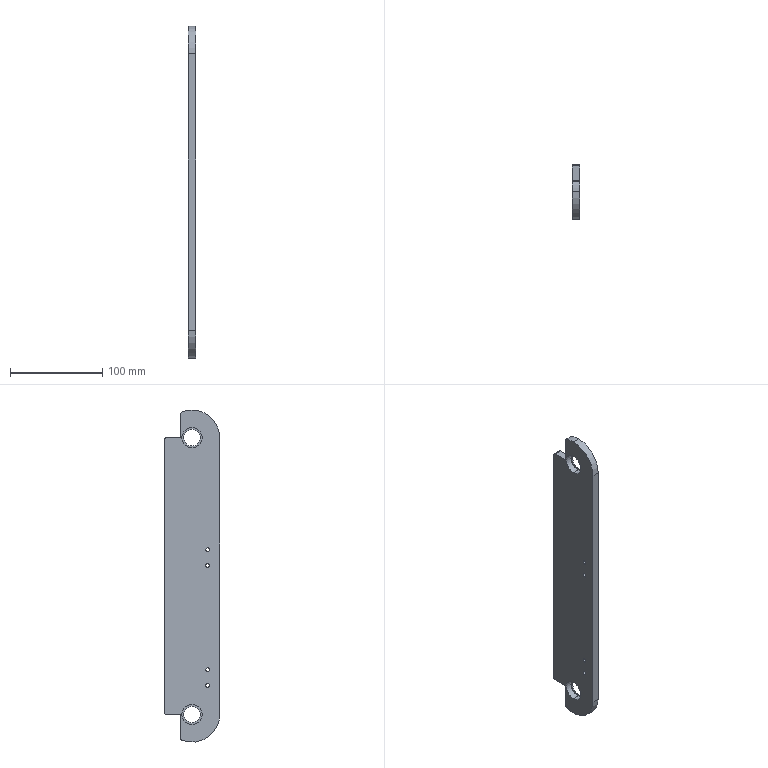Component | SolidWorks | ZHDJ-G001-2 | 1 solid | 33 faces | box 8 x 60 x 360 mm | volume 154619 mm3 | cylinder 23 | plane 10 | commonest cylinder face diameters 4.2 x8 18 x4 22 x4 4 x4 60 x3
STEP:
#1=COLOUR_RGB('',0.7922,0.8196,0.9333);
#2=FILL_AREA_STYLE_COLOUR('',#1);
#3=FILL_AREA_STYLE('',(#2));
#4=SURFACE_STYLE_FILL_AREA(#3);
#5=SURFACE_SIDE_STYLE('',(#4));
#6=SURFACE_STYLE_USAGE(.BOTH.,#5);
#7=PRESENTATION_STYLE_ASSIGNMENT((#6));
#8=CARTESIAN_POINT('',(1.772,-0.,-6.26));
#9=VERTEX_POINT('',#8);
#10=CARTESIAN_POINT('',(1.772,-0.,-5.551));
#11=VERTEX_POINT('',#10);
#12=CARTESIAN_POINT('',(1.772,-0.,-5.906));
#13=DIRECTION('',(-1.,0.,0.));
#14=DIRECTION('',(0.,0.,1.));
#15=AXIS2_PLACEMENT_3D('',#12,#13,#14);
#16=CIRCLE('',#15,0.3543);
#17=EDGE_CURVE('',#9,#11,#16,.T.);
#18=ORIENTED_EDGE('',*,*,#17,.T.);
#19=CARTESIAN_POINT('',(1.811,-0.,-5.551));
#20=VERTEX_POINT('',#19);
#21=CARTESIAN_POINT('',(1.417,-0.,-5.551));
#22=DIRECTION('',(1.,0.,0.));
#23=VECTOR('',#22,39.37);
#24=LINE('',#21,#23);
#25=EDGE_CURVE('',#11,#20,#24,.T.);
#26=ORIENTED_EDGE('',*,*,#25,.T.);
#27=CARTESIAN_POINT('',(1.811,-0.,-6.26));
#28=VERTEX_POINT('',#27);
#29=CARTESIAN_POINT('',(1.811,-0.,-5.906));
#30=DIRECTION('',(1.,0.,0.));
#31=DIRECTION('',(0.,0.,-1.));
#32=AXIS2_PLACEMENT_3D('',#29,#30,#31);
#33=CIRCLE('',#32,0.3543);
#34=EDGE_CURVE('',#20,#28,#33,.T.);
#35=ORIENTED_EDGE('',*,*,#34,.T.);
#36=CARTESIAN_POINT('',(1.417,-0.,-6.26));
#37=DIRECTION('',(1.,0.,0.));
#38=VECTOR('',#37,39.37);
#39=LINE('',#36,#38);
#40=EDGE_CURVE('',#9,#28,#39,.T.);
#41=ORIENTED_EDGE('',*,*,#40,.F.);
#42=EDGE_LOOP('',(#18,#26,#35,#41));
#43=FACE_OUTER_BOUND('',#42,.T.);
#44=CARTESIAN_POINT('',(1.417,-0.,-5.906));
#45=DIRECTION('',(1.,0.,0.));
#46=DIRECTION('',(0.,0.,-1.));
#47=AXIS2_PLACEMENT_3D('',#44,#45,#46);
#48=CYLINDRICAL_SURFACE('',#47,0.3543);
#49=ADVANCED_FACE('',(#43),#48,.F.);
#50=CARTESIAN_POINT('',(1.496,-0.6693,0.5354));
#51=VERTEX_POINT('',#50);
#52=CARTESIAN_POINT('',(1.496,-0.6693,0.3701));
#53=VERTEX_POINT('',#52);
#54=CARTESIAN_POINT('',(1.496,-0.6693,0.4528));
#55=DIRECTION('',(1.,0.,0.));
#56=DIRECTION('',(0.,0.,-1.));
#57=AXIS2_PLACEMENT_3D('',#54,#55,#56);
#58=CIRCLE('',#57,0.08268);
#59=EDGE_CURVE('',#51,#53,#58,.T.);
#60=ORIENTED_EDGE('',*,*,#59,.F.);
#61=CARTESIAN_POINT('',(1.811,-0.6693,0.5354));
#62=VERTEX_POINT('',#61);
#63=CARTESIAN_POINT('',(1.811,-0.6693,0.5354));
#64=DIRECTION('',(1.,0.,0.));
#65=VECTOR('',#64,39.37);
#66=LINE('',#63,#65);
#67=EDGE_CURVE('',#51,#62,#66,.T.);
#68=ORIENTED_EDGE('',*,*,#67,.T.);
#69=CARTESIAN_POINT('',(1.811,-0.6693,0.3701));
#70=VERTEX_POINT('',#69);
#71=CARTESIAN_POINT('',(1.811,-0.6693,0.4528));
#72=DIRECTION('',(1.,0.,0.));
#73=DIRECTION('',(0.,0.,-1.));
#74=AXIS2_PLACEMENT_3D('',#71,#72,#73);
#75=CIRCLE('',#74,0.08268);
#76=EDGE_CURVE('',#62,#70,#75,.T.);
#77=ORIENTED_EDGE('',*,*,#76,.T.);
#78=CARTESIAN_POINT('',(1.811,-0.6693,0.3701));
#79=DIRECTION('',(1.,0.,0.));
#80=VECTOR('',#79,39.37);
#81=LINE('',#78,#80);
#82=EDGE_CURVE('',#53,#70,#81,.T.);
#83=ORIENTED_EDGE('',*,*,#82,.F.);
#84=EDGE_LOOP('',(#60,#68,#77,#83));
#85=FACE_OUTER_BOUND('',#84,.T.);
#86=CARTESIAN_POINT('',(1.811,-0.6693,0.4528));
#87=DIRECTION('',(1.,0.,0.));
#88=DIRECTION('',(0.,0.,-1.));
#89=AXIS2_PLACEMENT_3D('',#86,#87,#88);
#90=CYLINDRICAL_SURFACE('',#89,0.08268);
#91=ADVANCED_FACE('',(#85),#90,.F.);
#92=CARTESIAN_POINT('',(1.496,-0.6693,1.205));
#93=VERTEX_POINT('',#92);
#94=CARTESIAN_POINT('',(1.496,-0.6693,1.039));
#95=VERTEX_POINT('',#94);
#96=CARTESIAN_POINT('',(1.496,-0.6693,1.122));
#97=DIRECTION('',(1.,0.,0.));
#98=DIRECTION('',(0.,0.,-1.));
#99=AXIS2_PLACEMENT_3D('',#96,#97,#98);
#100=CIRCLE('',#99,0.08268);
#101=EDGE_CURVE('',#93,#95,#100,.T.);
#102=ORIENTED_EDGE('',*,*,#101,.F.);
#103=CARTESIAN_POINT('',(1.811,-0.6693,1.205));
#104=VERTEX_POINT('',#103);
#105=CARTESIAN_POINT('',(1.811,-0.6693,1.205));
#106=DIRECTION('',(1.,0.,0.));
#107=VECTOR('',#106,39.37);
#108=LINE('',#105,#107);
#109=EDGE_CURVE('',#93,#104,#108,.T.);
#110=ORIENTED_EDGE('',*,*,#109,.T.);
#111=CARTESIAN_POINT('',(1.811,-0.6693,1.039));
#112=VERTEX_POINT('',#111);
#113=CARTESIAN_POINT('',(1.811,-0.6693,1.122));
#114=DIRECTION('',(1.,0.,0.));
#115=DIRECTION('',(0.,0.,-1.));
#116=AXIS2_PLACEMENT_3D('',#113,#114,#115);
#117=CIRCLE('',#116,0.08268);
#118=EDGE_CURVE('',#104,#112,#117,.T.);
#119=ORIENTED_EDGE('',*,*,#118,.T.);
#120=CARTESIAN_POINT('',(1.811,-0.6693,1.039));
#121=DIRECTION('',(1.,0.,0.));
#122=VECTOR('',#121,39.37);
#123=LINE('',#120,#122);
#124=EDGE_CURVE('',#95,#112,#123,.T.);
#125=ORIENTED_EDGE('',*,*,#124,.F.);
#126=EDGE_LOOP('',(#102,#110,#119,#125));
#127=FACE_OUTER_BOUND('',#126,.T.);
#128=CARTESIAN_POINT('',(1.811,-0.6693,1.122));
#129=DIRECTION('',(1.,0.,0.));
#130=DIRECTION('',(0.,0.,-1.));
#131=AXIS2_PLACEMENT_3D('',#128,#129,#130);
#132=CYLINDRICAL_SURFACE('',#131,0.08268);
#133=ADVANCED_FACE('',(#127),#132,.F.);
#134=CARTESIAN_POINT('',(1.496,-0.6693,-4.583));
#135=VERTEX_POINT('',#134);
#136=CARTESIAN_POINT('',(1.496,-0.6693,-4.748));
#137=VERTEX_POINT('',#136);
#138=CARTESIAN_POINT('',(1.496,-0.6693,-4.665));
#139=DIRECTION('',(1.,0.,0.));
#140=DIRECTION('',(0.,0.,-1.));
#141=AXIS2_PLACEMENT_3D('',#138,#139,#140);
#142=CIRCLE('',#141,0.08268);
#143=EDGE_CURVE('',#135,#137,#142,.T.);
#144=ORIENTED_EDGE('',*,*,#143,.F.);
#145=CARTESIAN_POINT('',(1.811,-0.6693,-4.583));
#146=VERTEX_POINT('',#145);
#147=CARTESIAN_POINT('',(1.811,-0.6693,-4.583));
#148=DIRECTION('',(1.,0.,0.));
#149=VECTOR('',#148,39.37);
#150=LINE('',#147,#149);
#151=EDGE_CURVE('',#135,#146,#150,.T.);
#152=ORIENTED_EDGE('',*,*,#151,.T.);
#153=CARTESIAN_POINT('',(1.811,-0.6693,-4.748));
#154=VERTEX_POINT('',#153);
#155=CARTESIAN_POINT('',(1.811,-0.6693,-4.665));
#156=DIRECTION('',(1.,0.,0.));
#157=DIRECTION('',(0.,0.,-1.));
#158=AXIS2_PLACEMENT_3D('',#155,#156,#157);
#159=CIRCLE('',#158,0.08268);
#160=EDGE_CURVE('',#146,#154,#159,.T.);
#161=ORIENTED_EDGE('',*,*,#160,.T.);
#162=CARTESIAN_POINT('',(1.811,-0.6693,-4.748));
#163=DIRECTION('',(1.,0.,0.));
#164=VECTOR('',#163,39.37);
#165=LINE('',#162,#164);
#166=EDGE_CURVE('',#137,#154,#165,.T.);
#167=ORIENTED_EDGE('',*,*,#166,.F.);
#168=EDGE_LOOP('',(#144,#152,#161,#167));
#169=FACE_OUTER_BOUND('',#168,.T.);
#170=CARTESIAN_POINT('',(1.811,-0.6693,-4.665));
#171=DIRECTION('',(1.,0.,0.));
#172=DIRECTION('',(0.,0.,-1.));
#173=AXIS2_PLACEMENT_3D('',#170,#171,#172);
#174=CYLINDRICAL_SURFACE('',#173,0.08268);
#175=ADVANCED_FACE('',(#169),#174,.F.);
#176=CARTESIAN_POINT('',(1.496,-0.6693,-3.913));
#177=VERTEX_POINT('',#176);
#178=CARTESIAN_POINT('',(1.496,-0.6693,-4.079));
#179=VERTEX_POINT('',#178);
#180=CARTESIAN_POINT('',(1.496,-0.6693,-3.996));
#181=DIRECTION('',(1.,0.,0.));
#182=DIRECTION('',(0.,0.,-1.));
#183=AXIS2_PLACEMENT_3D('',#180,#181,#182);
#184=CIRCLE('',#183,0.08268);
#185=EDGE_CURVE('',#177,#179,#184,.T.);
#186=ORIENTED_EDGE('',*,*,#185,.F.);
#187=CARTESIAN_POINT('',(1.811,-0.6693,-3.913));
#188=VERTEX_POINT('',#187);
#189=CARTESIAN_POINT('',(1.811,-0.6693,-3.913));
#190=DIRECTION('',(1.,0.,0.));
#191=VECTOR('',#190,39.37);
#192=LINE('',#189,#191);
#193=EDGE_CURVE('',#177,#188,#192,.T.);
#194=ORIENTED_EDGE('',*,*,#193,.T.);
#195=CARTESIAN_POINT('',(1.811,-0.6693,-4.079));
#196=VERTEX_POINT('',#195);
#197=CARTESIAN_POINT('',(1.811,-0.6693,-3.996));
#198=DIRECTION('',(1.,0.,0.));
#199=DIRECTION('',(0.,0.,-1.));
#200=AXIS2_PLACEMENT_3D('',#197,#198,#199);
#201=CIRCLE('',#200,0.08268);
#202=EDGE_CURVE('',#188,#196,#201,.T.);
#203=ORIENTED_EDGE('',*,*,#202,.T.);
#204=CARTESIAN_POINT('',(1.811,-0.6693,-4.079));
#205=DIRECTION('',(1.,0.,0.));
#206=VECTOR('',#205,39.37);
#207=LINE('',#204,#206);
#208=EDGE_CURVE('',#179,#196,#207,.T.);
#209=ORIENTED_EDGE('',*,*,#208,.F.);
#210=EDGE_LOOP('',(#186,#194,#203,#209));
#211=FACE_OUTER_BOUND('',#210,.T.);
#212=CARTESIAN_POINT('',(1.811,-0.6693,-3.996));
#213=DIRECTION('',(1.,0.,0.));
#214=DIRECTION('',(0.,0.,-1.));
#215=AXIS2_PLACEMENT_3D('',#212,#213,#214);
#216=CYLINDRICAL_SURFACE('',#215,0.08268);
#217=ADVANCED_FACE('',(#211),#216,.F.);
#218=CARTESIAN_POINT('',(1.772,0.,-5.472));
#219=VERTEX_POINT('',#218);
#220=CARTESIAN_POINT('',(1.772,0.,-6.339));
#221=VERTEX_POINT('',#220);
#222=CARTESIAN_POINT('',(1.772,0.,-5.906));
#223=DIRECTION('',(1.,0.,0.));
#224=DIRECTION('',(0.,0.,-1.));
#225=AXIS2_PLACEMENT_3D('',#222,#223,#224);
#226=CIRCLE('',#225,0.4331);
#227=EDGE_CURVE('',#219,#221,#226,.T.);
#228=ORIENTED_EDGE('',*,*,#227,.T.);
#229=CARTESIAN_POINT('',(1.496,0.,-6.339));
#230=VERTEX_POINT('',#229);
#231=CARTESIAN_POINT('',(1.772,0.,-6.339));
#232=DIRECTION('',(-1.,0.,0.));
#233=VECTOR('',#232,39.37);
#234=LINE('',#231,#233);
#235=EDGE_CURVE('',#221,#230,#234,.T.);
#236=ORIENTED_EDGE('',*,*,#235,.T.);
#237=CARTESIAN_POINT('',(1.496,0.,-5.472));
#238=VERTEX_POINT('',#237);
#239=CARTESIAN_POINT('',(1.496,0.,-5.906));
#240=DIRECTION('',(1.,0.,0.));
#241=DIRECTION('',(0.,0.,-1.));
#242=AXIS2_PLACEMENT_3D('',#239,#240,#241);
#243=CIRCLE('',#242,0.4331);
#244=EDGE_CURVE('',#238,#230,#243,.T.);
#245=ORIENTED_EDGE('',*,*,#244,.F.);
#246=CARTESIAN_POINT('',(1.772,0.,-5.472));
#247=DIRECTION('',(-1.,0.,0.));
#248=VECTOR('',#247,39.37);
#249=LINE('',#246,#248);
#250=EDGE_CURVE('',#219,#238,#249,.T.);
#251=ORIENTED_EDGE('',*,*,#250,.F.);
#252=EDGE_LOOP('',(#228,#236,#245,#251));
#253=FACE_OUTER_BOUND('',#252,.T.);
#254=CARTESIAN_POINT('',(1.772,0.,-5.906));
#255=DIRECTION('',(-1.,0.,0.));
#256=DIRECTION('',(0.,0.,1.));
#257=AXIS2_PLACEMENT_3D('',#254,#255,#256);
#258=CYLINDRICAL_SURFACE('',#257,0.4331);
#259=ADVANCED_FACE('',(#253),#258,.F.);
#260=CARTESIAN_POINT('',(1.772,0.,5.472));
#261=VERTEX_POINT('',#260);
#262=CARTESIAN_POINT('',(1.772,0.,6.339));
#263=VERTEX_POINT('',#262);
#264=CARTESIAN_POINT('',(1.772,0.,5.906));
#265=DIRECTION('',(-1.,0.,0.));
#266=DIRECTION('',(0.,0.,1.));
#267=AXIS2_PLACEMENT_3D('',#264,#265,#266);
#268=CIRCLE('',#267,0.4331);
#269=EDGE_CURVE('',#261,#263,#268,.T.);
#270=ORIENTED_EDGE('',*,*,#269,.F.);
#271=CARTESIAN_POINT('',(1.496,0.,5.472));
#272=VERTEX_POINT('',#271);
#273=CARTESIAN_POINT('',(1.772,0.,5.472));
#274=DIRECTION('',(-1.,0.,0.));
#275=VECTOR('',#274,39.37);
#276=LINE('',#273,#275);
#277=EDGE_CURVE('',#261,#272,#276,.T.);
#278=ORIENTED_EDGE('',*,*,#277,.T.);
#279=CARTESIAN_POINT('',(1.496,0.,6.339));
#280=VERTEX_POINT('',#279);
#281=CARTESIAN_POINT('',(1.496,0.,5.906));
#282=DIRECTION('',(-1.,0.,0.));
#283=DIRECTION('',(0.,0.,1.));
#284=AXIS2_PLACEMENT_3D('',#281,#282,#283);
#285=CIRCLE('',#284,0.4331);
#286=EDGE_CURVE('',#272,#280,#285,.T.);
#287=ORIENTED_EDGE('',*,*,#286,.T.);
#288=CARTESIAN_POINT('',(1.772,0.,6.339));
#289=DIRECTION('',(-1.,0.,0.));
#290=VECTOR('',#289,39.37);
#291=LINE('',#288,#290);
#292=EDGE_CURVE('',#263,#280,#291,.T.);
#293=ORIENTED_EDGE('',*,*,#292,.F.);
#294=EDGE_LOOP('',(#270,#278,#287,#293));
#295=FACE_OUTER_BOUND('',#294,.T.);
#296=CARTESIAN_POINT('',(1.772,0.,5.906));
#297=DIRECTION('',(-1.,0.,0.));
#298=DIRECTION('',(0.,0.,1.));
#299=AXIS2_PLACEMENT_3D('',#296,#297,#298);
#300=CYLINDRICAL_SURFACE('',#299,0.4331);
#301=ADVANCED_FACE('',(#295),#300,.F.);
#302=CARTESIAN_POINT('',(1.811,-0.,7.087));
#303=VERTEX_POINT('',#302);
#304=CARTESIAN_POINT('',(1.811,-1.181,5.906));
#305=VERTEX_POINT('',#304);
#306=CARTESIAN_POINT('',(1.811,-0.,5.906));
#307=DIRECTION('',(1.,0.,0.));
#308=DIRECTION('',(0.,0.,-1.));
#309=AXIS2_PLACEMENT_3D('',#306,#307,#308);
#310=CIRCLE('',#309,1.181);
#311=EDGE_CURVE('',#303,#305,#310,.T.);
#312=ORIENTED_EDGE('',*,*,#311,.F.);
#313=CARTESIAN_POINT('',(1.496,-0.,7.087));
#314=VERTEX_POINT('',#313);
#315=CARTESIAN_POINT('',(1.811,-0.,7.087));
#316=DIRECTION('',(-1.,0.,0.));
#317=VECTOR('',#316,39.37);
#318=LINE('',#315,#317);
#319=EDGE_CURVE('',#303,#314,#318,.T.);
#320=ORIENTED_EDGE('',*,*,#319,.T.);
#321=CARTESIAN_POINT('',(1.496,-1.181,5.906));
#322=VERTEX_POINT('',#321);
#323=CARTESIAN_POINT('',(1.496,-0.,5.906));
#324=DIRECTION('',(1.,0.,0.));
#325=DIRECTION('',(0.,0.,-1.));
#326=AXIS2_PLACEMENT_3D('',#323,#324,#325);
#327=CIRCLE('',#326,1.181);
#328=EDGE_CURVE('',#314,#322,#327,.T.);
#329=ORIENTED_EDGE('',*,*,#328,.T.);
#330=CARTESIAN_POINT('',(1.811,-1.181,5.906));
#331=DIRECTION('',(-1.,0.,0.));
#332=VECTOR('',#331,39.37);
#333=LINE('',#330,#332);
#334=EDGE_CURVE('',#305,#322,#333,.T.);
#335=ORIENTED_EDGE('',*,*,#334,.F.);
#336=EDGE_LOOP('',(#312,#320,#329,#335));
#337=FACE_OUTER_BOUND('',#336,.T.);
#338=CARTESIAN_POINT('',(1.811,-0.,5.906));
#339=DIRECTION('',(-1.,0.,0.));
#340=DIRECTION('',(0.,0.,1.));
#341=AXIS2_PLACEMENT_3D('',#338,#339,#340);
#342=CYLINDRICAL_SURFACE('',#341,1.181);
#343=ADVANCED_FACE('',(#337),#342,.T.);
#344=CARTESIAN_POINT('',(1.772,0.,6.26));
#345=VERTEX_POINT('',#344);
#346=CARTESIAN_POINT('',(1.772,0.,5.551));
#347=VERTEX_POINT('',#346);
#348=CARTESIAN_POINT('',(1.772,0.,5.906));
#349=DIRECTION('',(1.,0.,0.));
#350=DIRECTION('',(0.,0.,1.));
#351=AXIS2_PLACEMENT_3D('',#348,#349,#350);
#352=CIRCLE('',#351,0.3543);
#353=EDGE_CURVE('',#345,#347,#352,.T.);
#354=ORIENTED_EDGE('',*,*,#353,.F.);
#355=CARTESIAN_POINT('',(1.811,0.,6.26));
#356=VERTEX_POINT('',#355);
#357=CARTESIAN_POINT('',(1.417,0.,6.26));
#358=DIRECTION('',(1.,0.,0.));
#359=VECTOR('',#358,39.37);
#360=LINE('',#357,#359);
#361=EDGE_CURVE('',#345,#356,#360,.T.);
#362=ORIENTED_EDGE('',*,*,#361,.T.);
#363=CARTESIAN_POINT('',(1.811,0.,5.551));
#364=VERTEX_POINT('',#363);
#365=CARTESIAN_POINT('',(1.811,0.,5.906));
#366=DIRECTION('',(1.,0.,0.));
#367=DIRECTION('',(0.,0.,-1.));
#368=AXIS2_PLACEMENT_3D('',#365,#366,#367);
#369=CIRCLE('',#368,0.3543);
#370=EDGE_CURVE('',#356,#364,#369,.T.);
#371=ORIENTED_EDGE('',*,*,#370,.T.);
#372=CARTESIAN_POINT('',(1.417,0.,5.551));
#373=DIRECTION('',(1.,0.,0.));
#374=VECTOR('',#373,39.37);
#375=LINE('',#372,#374);
#376=EDGE_CURVE('',#347,#364,#375,.T.);
#377=ORIENTED_EDGE('',*,*,#376,.F.);
#378=EDGE_LOOP('',(#354,#362,#371,#377));
#379=FACE_OUTER_BOUND('',#378,.T.);
#380=CARTESIAN_POINT('',(1.417,0.,5.906));
#381=DIRECTION('',(1.,0.,0.));
#382=DIRECTION('',(0.,0.,-1.));
#383=AXIS2_PLACEMENT_3D('',#380,#381,#382);
#384=CYLINDRICAL_SURFACE('',#383,0.3543);
#385=ADVANCED_FACE('',(#379),#384,.F.);
#386=CARTESIAN_POINT('',(1.496,-1.181,-5.906));
#387=VERTEX_POINT('',#386);
#388=CARTESIAN_POINT('',(1.496,0.4218,-7.009));
#389=VERTEX_POINT('',#388);
#390=CARTESIAN_POINT('',(1.496,-0.,-5.906));
#391=DIRECTION('',(1.,0.,0.));
#392=DIRECTION('',(0.,0.,-1.));
#393=AXIS2_PLACEMENT_3D('',#390,#391,#392);
#394=CIRCLE('',#393,1.181);
#395=EDGE_CURVE('',#387,#389,#394,.T.);
#396=ORIENTED_EDGE('',*,*,#395,.T.);
#397=CARTESIAN_POINT('',(1.811,0.4218,-7.009));
#398=VERTEX_POINT('',#397);
#399=CARTESIAN_POINT('',(1.811,0.4218,-7.009));
#400=DIRECTION('',(1.,0.,0.));
#401=VECTOR('',#400,39.37);
#402=LINE('',#399,#401);
#403=EDGE_CURVE('',#389,#398,#402,.T.);
#404=ORIENTED_EDGE('',*,*,#403,.T.);
#405=CARTESIAN_POINT('',(1.811,-1.181,-5.906));
#406=VERTEX_POINT('',#405);
#407=CARTESIAN_POINT('',(1.811,-0.,-5.906));
#408=DIRECTION('',(1.,0.,0.));
#409=DIRECTION('',(0.,0.,-1.));
#410=AXIS2_PLACEMENT_3D('',#407,#408,#409);
#411=CIRCLE('',#410,1.181);
#412=EDGE_CURVE('',#406,#398,#411,.T.);
#413=ORIENTED_EDGE('',*,*,#412,.F.);
#414=CARTESIAN_POINT('',(1.811,-1.181,-5.906));
#415=DIRECTION('',(-1.,0.,0.));
#416=VECTOR('',#415,39.37);
#417=LINE('',#414,#416);
#418=EDGE_CURVE('',#406,#387,#417,.T.);
#419=ORIENTED_EDGE('',*,*,#418,.T.);
#420=EDGE_LOOP('',(#396,#404,#413,#419));
#421=FACE_OUTER_BOUND('',#420,.T.);
#422=CARTESIAN_POINT('',(1.811,-0.,-5.906));
#423=DIRECTION('',(-1.,0.,0.));
#424=DIRECTION('',(0.,0.,1.));
#425=AXIS2_PLACEMENT_3D('',#422,#423,#424);
#426=CYLINDRICAL_SURFACE('',#425,1.181);
#427=ADVANCED_FACE('',(#421),#426,.T.);
#428=CARTESIAN_POINT('',(1.811,-0.,-5.906));
#429=DIRECTION('',(1.,0.,0.));
#430=DIRECTION('',(0.,0.,-1.));
#431=AXIS2_PLACEMENT_3D('',#428,#429,#430);
#432=CIRCLE('',#431,0.3543);
#433=EDGE_CURVE('',#28,#20,#432,.T.);
#434=ORIENTED_EDGE('',*,*,#433,.F.);
#435=ORIENTED_EDGE('',*,*,#34,.F.);
#436=EDGE_LOOP('',(#434,#435));
#437=FACE_BOUND('',#436,.T.);
#438=CARTESIAN_POINT('',(1.811,-0.6693,0.4528));
#439=DIRECTION('',(1.,0.,0.));
#440=DIRECTION('',(0.,0.,-1.));
#441=AXIS2_PLACEMENT_3D('',#438,#439,#440);
#442=CIRCLE('',#441,0.08268);
#443=EDGE_CURVE('',#70,#62,#442,.T.);
#444=ORIENTED_EDGE('',*,*,#443,.F.);
#445=ORIENTED_EDGE('',*,*,#76,.F.);
#446=EDGE_LOOP('',(#444,#445));
#447=FACE_BOUND('',#446,.T.);
#448=CARTESIAN_POINT('',(1.811,-0.6693,1.122));
#449=DIRECTION('',(1.,0.,0.));
#450=DIRECTION('',(0.,0.,-1.));
#451=AXIS2_PLACEMENT_3D('',#448,#449,#450);
#452=CIRCLE('',#451,0.08268);
#453=EDGE_CURVE('',#112,#104,#452,.T.);
#454=ORIENTED_EDGE('',*,*,#453,.F.);
#455=ORIENTED_EDGE('',*,*,#118,.F.);
#456=EDGE_LOOP('',(#454,#455));
#457=FACE_BOUND('',#456,.T.);
#458=CARTESIAN_POINT('',(1.811,-0.6693,-4.665));
#459=DIRECTION('',(1.,0.,0.));
#460=DIRECTION('',(0.,0.,-1.));
#461=AXIS2_PLACEMENT_3D('',#458,#459,#460);
#462=CIRCLE('',#461,0.08268);
#463=EDGE_CURVE('',#154,#146,#462,.T.);
#464=ORIENTED_EDGE('',*,*,#463,.F.);
#465=ORIENTED_EDGE('',*,*,#160,.F.);
#466=EDGE_LOOP('',(#464,#465));
#467=FACE_BOUND('',#466,.T.);
#468=CARTESIAN_POINT('',(1.811,-0.6693,-3.996));
#469=DIRECTION('',(1.,0.,0.));
#470=DIRECTION('',(0.,0.,-1.));
#471=AXIS2_PLACEMENT_3D('',#468,#469,#470);
#472=CIRCLE('',#471,0.08268);
#473=EDGE_CURVE('',#196,#188,#472,.T.);
#474=ORIENTED_EDGE('',*,*,#473,.F.);
#475=ORIENTED_EDGE('',*,*,#202,.F.);
#476=EDGE_LOOP('',(#474,#475));
#477=FACE_BOUND('',#476,.T.);
#478=CARTESIAN_POINT('',(1.811,0.,5.906));
#479=DIRECTION('',(1.,0.,0.));
#480=DIRECTION('',(0.,0.,-1.));
#481=AXIS2_PLACEMENT_3D('',#478,#479,#480);
#482=CIRCLE('',#481,0.3543);
#483=EDGE_CURVE('',#364,#356,#482,.T.);
#484=ORIENTED_EDGE('',*,*,#483,.F.);
#485=ORIENTED_EDGE('',*,*,#370,.F.);
#486=EDGE_LOOP('',(#484,#485));
#487=FACE_BOUND('',#486,.T.);
#488=ORIENTED_EDGE('',*,*,#412,.T.);
#489=CARTESIAN_POINT('',(1.811,0.4724,-6.935));
#490=VERTEX_POINT('',#489);
#491=CARTESIAN_POINT('',(1.811,0.3937,-6.935));
#492=DIRECTION('',(1.,0.,0.));
#493=DIRECTION('',(0.,0.,-1.));
#494=AXIS2_PLACEMENT_3D('',#491,#492,#493);
#495=CIRCLE('',#494,0.07874);
#496=EDGE_CURVE('',#398,#490,#495,.T.);
#497=ORIENTED_EDGE('',*,*,#496,.T.);
#498=CARTESIAN_POINT('',(1.811,0.4724,-5.906));
#499=VERTEX_POINT('',#498);
#500=CARTESIAN_POINT('',(1.811,0.4724,-5.906));
#501=DIRECTION('',(0.,0.,1.));
#502=VECTOR('',#501,39.37);
#503=LINE('',#500,#502);
#504=EDGE_CURVE('',#490,#499,#503,.T.);
#505=ORIENTED_EDGE('',*,*,#504,.T.);
#506=CARTESIAN_POINT('',(1.811,1.102,-5.906));
#507=VERTEX_POINT('',#506);
#508=CARTESIAN_POINT('',(1.811,1.181,-5.906));
#509=DIRECTION('',(0.,1.,0.));
#510=VECTOR('',#509,39.37);
#511=LINE('',#508,#510);
#512=EDGE_CURVE('',#499,#507,#511,.T.);
#513=ORIENTED_EDGE('',*,*,#512,.T.);
#514=CARTESIAN_POINT('',(1.811,1.181,-5.827));
#515=VERTEX_POINT('',#514);
#516=CARTESIAN_POINT('',(1.811,1.102,-5.827));
#517=DIRECTION('',(1.,0.,0.));
#518=DIRECTION('',(0.,0.,-1.));
#519=AXIS2_PLACEMENT_3D('',#516,#517,#518);
#520=CIRCLE('',#519,0.07874);
#521=EDGE_CURVE('',#507,#515,#520,.T.);
#522=ORIENTED_EDGE('',*,*,#521,.T.);
#523=CARTESIAN_POINT('',(1.811,1.181,5.827));
#524=VERTEX_POINT('',#523);
#525=CARTESIAN_POINT('',(1.811,1.181,5.906));
#526=DIRECTION('',(0.,-0.,1.));
#527=VECTOR('',#526,39.37);
#528=LINE('',#525,#527);
#529=EDGE_CURVE('',#515,#524,#528,.T.);
#530=ORIENTED_EDGE('',*,*,#529,.T.);
#531=CARTESIAN_POINT('',(1.811,1.102,5.906));
#532=VERTEX_POINT('',#531);
#533=CARTESIAN_POINT('',(1.811,1.102,5.827));
#534=DIRECTION('',(1.,0.,0.));
#535=DIRECTION('',(0.,0.,-1.));
#536=AXIS2_PLACEMENT_3D('',#533,#534,#535);
#537=CIRCLE('',#536,0.07874);
#538=EDGE_CURVE('',#524,#532,#537,.T.);
#539=ORIENTED_EDGE('',*,*,#538,.T.);
#540=CARTESIAN_POINT('',(1.811,0.4724,5.906));
#541=VERTEX_POINT('',#540);
#542=CARTESIAN_POINT('',(1.811,1.181,5.906));
#543=DIRECTION('',(0.,1.,0.));
#544=VECTOR('',#543,39.37);
#545=LINE('',#542,#544);
#546=EDGE_CURVE('',#541,#532,#545,.T.);
#547=ORIENTED_EDGE('',*,*,#546,.F.);
#548=CARTESIAN_POINT('',(1.811,0.4724,6.935));
#549=VERTEX_POINT('',#548);
#550=CARTESIAN_POINT('',(1.811,0.4724,5.906));
#551=DIRECTION('',(0.,0.,-1.));
#552=VECTOR('',#551,39.37);
#553=LINE('',#550,#552);
#554=EDGE_CURVE('',#549,#541,#553,.T.);
#555=ORIENTED_EDGE('',*,*,#554,.F.);
#556=CARTESIAN_POINT('',(1.811,0.4218,7.009));
#557=VERTEX_POINT('',#556);
#558=CARTESIAN_POINT('',(1.811,0.3937,6.935));
#559=DIRECTION('',(1.,0.,0.));
#560=DIRECTION('',(0.,0.,-1.));
#561=AXIS2_PLACEMENT_3D('',#558,#559,#560);
#562=CIRCLE('',#561,0.07874);
#563=EDGE_CURVE('',#549,#557,#562,.T.);
#564=ORIENTED_EDGE('',*,*,#563,.T.);
#565=CARTESIAN_POINT('',(1.811,-0.,5.906));
#566=DIRECTION('',(1.,0.,0.));
#567=DIRECTION('',(0.,0.,-1.));
#568=AXIS2_PLACEMENT_3D('',#565,#566,#567);
#569=CIRCLE('',#568,1.181);
#570=EDGE_CURVE('',#557,#303,#569,.T.);
#571=ORIENTED_EDGE('',*,*,#570,.T.);
#572=ORIENTED_EDGE('',*,*,#311,.T.);
#573=CARTESIAN_POINT('',(1.811,-1.181,5.906));
#574=DIRECTION('',(0.,0.,-1.));
#575=VECTOR('',#574,39.37);
#576=LINE('',#573,#575);
#577=EDGE_CURVE('',#305,#406,#576,.T.);
#578=ORIENTED_EDGE('',*,*,#577,.T.);
#579=EDGE_LOOP('',(#488,#497,#505,#513,#522,#530,#539,#547,#555,#564,#571,#572,#578));
#580=FACE_OUTER_BOUND('',#579,.T.);
#581=CARTESIAN_POINT('',(1.811,-0.,5.906));
#582=DIRECTION('',(1.,0.,0.));
#583=DIRECTION('',(0.,0.,-1.));
#584=AXIS2_PLACEMENT_3D('',#581,#582,#583);
#585=PLANE('',#584);
#586=ADVANCED_FACE('',(#437,#447,#457,#467,#477,#487,#580),#585,.T.);
#587=CARTESIAN_POINT('',(1.496,0.,5.906));
#588=DIRECTION('',(-1.,0.,0.));
#589=DIRECTION('',(0.,0.,1.));
#590=AXIS2_PLACEMENT_3D('',#587,#588,#589);
#591=CIRCLE('',#590,0.4331);
#592=EDGE_CURVE('',#280,#272,#591,.T.);
#593=ORIENTED_EDGE('',*,*,#592,.F.);
#594=ORIENTED_EDGE('',*,*,#286,.F.);
#595=EDGE_LOOP('',(#593,#594));
#596=FACE_BOUND('',#595,.T.);
#597=ORIENTED_EDGE('',*,*,#244,.T.);
#598=CARTESIAN_POINT('',(1.496,0.,-5.906));
#599=DIRECTION('',(1.,0.,0.));
#600=DIRECTION('',(0.,0.,-1.));
#601=AXIS2_PLACEMENT_3D('',#598,#599,#600);
#602=CIRCLE('',#601,0.4331);
#603=EDGE_CURVE('',#230,#238,#602,.T.);
#604=ORIENTED_EDGE('',*,*,#603,.T.);
#605=EDGE_LOOP('',(#597,#604));
#606=FACE_BOUND('',#605,.T.);
#607=CARTESIAN_POINT('',(1.496,-0.6693,-3.996));
#608=DIRECTION('',(1.,0.,0.));
#609=DIRECTION('',(0.,0.,-1.));
#610=AXIS2_PLACEMENT_3D('',#607,#608,#609);
#611=CIRCLE('',#610,0.08268);
#612=EDGE_CURVE('',#179,#177,#611,.T.);
#613=ORIENTED_EDGE('',*,*,#612,.T.);
#614=ORIENTED_EDGE('',*,*,#185,.T.);
#615=EDGE_LOOP('',(#613,#614));
#616=FACE_BOUND('',#615,.T.);
#617=CARTESIAN_POINT('',(1.496,-0.6693,-4.665));
#618=DIRECTION('',(1.,0.,0.));
#619=DIRECTION('',(0.,0.,-1.));
#620=AXIS2_PLACEMENT_3D('',#617,#618,#619);
#621=CIRCLE('',#620,0.08268);
#622=EDGE_CURVE('',#137,#135,#621,.T.);
#623=ORIENTED_EDGE('',*,*,#622,.T.);
#624=ORIENTED_EDGE('',*,*,#143,.T.);
#625=EDGE_LOOP('',(#623,#624));
#626=FACE_BOUND('',#625,.T.);
#627=CARTESIAN_POINT('',(1.496,-0.6693,1.122));
#628=DIRECTION('',(1.,0.,0.));
#629=DIRECTION('',(0.,0.,-1.));
#630=AXIS2_PLACEMENT_3D('',#627,#628,#629);
#631=CIRCLE('',#630,0.08268);
#632=EDGE_CURVE('',#95,#93,#631,.T.);
#633=ORIENTED_EDGE('',*,*,#632,.T.);
#634=ORIENTED_EDGE('',*,*,#101,.T.);
#635=EDGE_LOOP('',(#633,#634));
#636=FACE_BOUND('',#635,.T.);
#637=CARTESIAN_POINT('',(1.496,-0.6693,0.4528));
#638=DIRECTION('',(1.,0.,0.));
#639=DIRECTION('',(0.,0.,-1.));
#640=AXIS2_PLACEMENT_3D('',#637,#638,#639);
#641=CIRCLE('',#640,0.08268);
#642=EDGE_CURVE('',#53,#51,#641,.T.);
#643=ORIENTED_EDGE('',*,*,#642,.T.);
#644=ORIENTED_EDGE('',*,*,#59,.T.);
#645=EDGE_LOOP('',(#643,#644));
#646=FACE_BOUND('',#645,.T.);
#647=CARTESIAN_POINT('',(1.496,0.4724,-6.935));
#648=VERTEX_POINT('',#647);
#649=CARTESIAN_POINT('',(1.496,0.4724,-5.906));
#650=VERTEX_POINT('',#649);
#651=CARTESIAN_POINT('',(1.496,0.4724,5.906));
#652=DIRECTION('',(0.,0.,1.));
#653=VECTOR('',#652,39.37);
#654=LINE('',#651,#653);
#655=EDGE_CURVE('',#648,#650,#654,.T.);
#656=ORIENTED_EDGE('',*,*,#655,.F.);
#657=CARTESIAN_POINT('',(1.496,0.3937,-6.935));
#658=DIRECTION('',(-1.,0.,0.));
#659=DIRECTION('',(0.,0.,-1.));
#660=AXIS2_PLACEMENT_3D('',#657,#658,#659);
#661=CIRCLE('',#660,0.07874);
#662=EDGE_CURVE('',#648,#389,#661,.T.);
#663=ORIENTED_EDGE('',*,*,#662,.T.);
#664=ORIENTED_EDGE('',*,*,#395,.F.);
#665=CARTESIAN_POINT('',(1.496,-1.181,5.906));
#666=DIRECTION('',(0.,0.,-1.));
#667=VECTOR('',#666,39.37);
#668=LINE('',#665,#667);
#669=EDGE_CURVE('',#322,#387,#668,.T.);
#670=ORIENTED_EDGE('',*,*,#669,.F.);
#671=ORIENTED_EDGE('',*,*,#328,.F.);
#672=CARTESIAN_POINT('',(1.496,0.4218,7.009));
#673=VERTEX_POINT('',#672);
#674=CARTESIAN_POINT('',(1.496,-0.,5.906));
#675=DIRECTION('',(1.,0.,0.));
#676=DIRECTION('',(0.,0.,-1.));
#677=AXIS2_PLACEMENT_3D('',#674,#675,#676);
#678=CIRCLE('',#677,1.181);
#679=EDGE_CURVE('',#673,#314,#678,.T.);
#680=ORIENTED_EDGE('',*,*,#679,.F.);
#681=CARTESIAN_POINT('',(1.496,0.4724,6.935));
#682=VERTEX_POINT('',#681);
#683=CARTESIAN_POINT('',(1.496,0.3937,6.935));
#684=DIRECTION('',(-1.,0.,0.));
#685=DIRECTION('',(0.,0.,-1.));
#686=AXIS2_PLACEMENT_3D('',#683,#684,#685);
#687=CIRCLE('',#686,0.07874);
#688=EDGE_CURVE('',#673,#682,#687,.T.);
#689=ORIENTED_EDGE('',*,*,#688,.T.);
#690=CARTESIAN_POINT('',(1.496,0.4724,5.906));
#691=VERTEX_POINT('',#690);
#692=CARTESIAN_POINT('',(1.496,0.4724,5.906));
#693=DIRECTION('',(0.,0.,-1.));
#694=VECTOR('',#693,39.37);
#695=LINE('',#692,#694);
#696=EDGE_CURVE('',#682,#691,#695,.T.);
#697=ORIENTED_EDGE('',*,*,#696,.T.);
#698=CARTESIAN_POINT('',(1.496,1.102,5.906));
#699=VERTEX_POINT('',#698);
#700=CARTESIAN_POINT('',(1.496,-0.,5.906));
#701=DIRECTION('',(0.,1.,0.));
#702=VECTOR('',#701,39.37);
#703=LINE('',#700,#702);
#704=EDGE_CURVE('',#691,#699,#703,.T.);
#705=ORIENTED_EDGE('',*,*,#704,.T.);
#706=CARTESIAN_POINT('',(1.496,1.181,5.827));
#707=VERTEX_POINT('',#706);
#708=CARTESIAN_POINT('',(1.496,1.102,5.827));
#709=DIRECTION('',(-1.,0.,0.));
#710=DIRECTION('',(0.,0.,-1.));
#711=AXIS2_PLACEMENT_3D('',#708,#709,#710);
#712=CIRCLE('',#711,0.07874);
#713=EDGE_CURVE('',#699,#707,#712,.T.);
#714=ORIENTED_EDGE('',*,*,#713,.T.);
#715=CARTESIAN_POINT('',(1.496,1.181,-5.827));
#716=VERTEX_POINT('',#715);
#717=CARTESIAN_POINT('',(1.496,1.181,5.906));
#718=DIRECTION('',(0.,-0.,1.));
#719=VECTOR('',#718,39.37);
#720=LINE('',#717,#719);
#721=EDGE_CURVE('',#716,#707,#720,.T.);
#722=ORIENTED_EDGE('',*,*,#721,.F.);
#723=CARTESIAN_POINT('',(1.496,1.102,-5.906));
#724=VERTEX_POINT('',#723);
#725=CARTESIAN_POINT('',(1.496,1.102,-5.827));
#726=DIRECTION('',(-1.,0.,0.));
#727=DIRECTION('',(0.,0.,-1.));
#728=AXIS2_PLACEMENT_3D('',#725,#726,#727);
#729=CIRCLE('',#728,0.07874);
#730=EDGE_CURVE('',#716,#724,#729,.T.);
#731=ORIENTED_EDGE('',*,*,#730,.T.);
#732=CARTESIAN_POINT('',(1.496,-0.,-5.906));
#733=DIRECTION('',(0.,1.,0.));
#734=VECTOR('',#733,39.37);
#735=LINE('',#732,#734);
#736=EDGE_CURVE('',#650,#724,#735,.T.);
#737=ORIENTED_EDGE('',*,*,#736,.F.);
#738=EDGE_LOOP('',(#656,#663,#664,#670,#671,#680,#689,#697,#705,#714,#722,#731,#737));
#739=FACE_OUTER_BOUND('',#738,.T.);
#740=CARTESIAN_POINT('',(1.496,-0.,5.906));
#741=DIRECTION('',(1.,0.,0.));
#742=DIRECTION('',(0.,0.,-1.));
#743=AXIS2_PLACEMENT_3D('',#740,#741,#742);
#744=PLANE('',#743);
#745=ADVANCED_FACE('',(#596,#606,#616,#626,#636,#646,#739),#744,.F.);
#746=ORIENTED_EDGE('',*,*,#361,.F.);
#747=CARTESIAN_POINT('',(1.772,0.,5.906));
#748=DIRECTION('',(1.,0.,0.));
#749=DIRECTION('',(0.,0.,1.));
#750=AXIS2_PLACEMENT_3D('',#747,#748,#749);
#751=CIRCLE('',#750,0.3543);
#752=EDGE_CURVE('',#347,#345,#751,.T.);
#753=ORIENTED_EDGE('',*,*,#752,.F.);
#754=ORIENTED_EDGE('',*,*,#376,.T.);
#755=ORIENTED_EDGE('',*,*,#483,.T.);
#756=EDGE_LOOP('',(#746,#753,#754,#755));
#757=FACE_OUTER_BOUND('',#756,.T.);
#758=CARTESIAN_POINT('',(1.417,0.,5.906));
#759=DIRECTION('',(1.,0.,0.));
#760=DIRECTION('',(0.,0.,-1.));
#761=AXIS2_PLACEMENT_3D('',#758,#759,#760);
#762=CYLINDRICAL_SURFACE('',#761,0.3543);
#763=ADVANCED_FACE('',(#757),#762,.F.);
#764=ORIENTED_EDGE('',*,*,#319,.F.);
#765=ORIENTED_EDGE('',*,*,#570,.F.);
#766=CARTESIAN_POINT('',(1.811,0.4218,7.009));
#767=DIRECTION('',(-1.,0.,0.));
#768=VECTOR('',#767,39.37);
#769=LINE('',#766,#768);
#770=EDGE_CURVE('',#557,#673,#769,.T.);
#771=ORIENTED_EDGE('',*,*,#770,.T.);
#772=ORIENTED_EDGE('',*,*,#679,.T.);
#773=EDGE_LOOP('',(#764,#765,#771,#772));
#774=FACE_OUTER_BOUND('',#773,.T.);
#775=CARTESIAN_POINT('',(1.811,-0.,5.906));
#776=DIRECTION('',(-1.,0.,0.));
#777=DIRECTION('',(0.,0.,1.));
#778=AXIS2_PLACEMENT_3D('',#775,#776,#777);
#779=CYLINDRICAL_SURFACE('',#778,1.181);
#780=ADVANCED_FACE('',(#774),#779,.T.);
#781=ORIENTED_EDGE('',*,*,#669,.T.);
#782=ORIENTED_EDGE('',*,*,#418,.F.);
#783=ORIENTED_EDGE('',*,*,#577,.F.);
#784=ORIENTED_EDGE('',*,*,#334,.T.);
#785=EDGE_LOOP('',(#781,#782,#783,#784));
#786=FACE_OUTER_BOUND('',#785,.T.);
#787=CARTESIAN_POINT('',(1.811,-1.181,5.906));
#788=DIRECTION('',(0.,1.,0.));
#789=DIRECTION('',(0.,0.,1.));
#790=AXIS2_PLACEMENT_3D('',#787,#788,#789);
#791=PLANE('',#790);
#792=ADVANCED_FACE('',(#786),#791,.F.);
#793=ORIENTED_EDGE('',*,*,#529,.F.);
#794=CARTESIAN_POINT('',(1.496,1.181,-5.827));
#795=DIRECTION('',(-1.,0.,0.));
#796=VECTOR('',#795,39.37);
#797=LINE('',#794,#796);
#798=EDGE_CURVE('',#515,#716,#797,.T.);
#799=ORIENTED_EDGE('',*,*,#798,.T.);
#800=ORIENTED_EDGE('',*,*,#721,.T.);
#801=CARTESIAN_POINT('',(1.811,1.181,5.827));
#802=DIRECTION('',(1.,0.,0.));
#803=VECTOR('',#802,39.37);
#804=LINE('',#801,#803);
#805=EDGE_CURVE('',#707,#524,#804,.T.);
#806=ORIENTED_EDGE('',*,*,#805,.T.);
#807=EDGE_LOOP('',(#793,#799,#800,#806));
#808=FACE_OUTER_BOUND('',#807,.T.);
#809=CARTESIAN_POINT('',(1.811,1.181,5.906));
#810=DIRECTION('',(0.,-1.,-0.));
#811=DIRECTION('',(0.,0.,-1.));
#812=AXIS2_PLACEMENT_3D('',#809,#810,#811);
#813=PLANE('',#812);
#814=ADVANCED_FACE('',(#808),#813,.F.);
#815=ORIENTED_EDGE('',*,*,#546,.T.);
#816=CARTESIAN_POINT('',(1.024,1.102,5.906));
#817=DIRECTION('',(-1.,0.,0.));
#818=VECTOR('',#817,39.37);
#819=LINE('',#816,#818);
#820=EDGE_CURVE('',#532,#699,#819,.T.);
#821=ORIENTED_EDGE('',*,*,#820,.T.);
#822=ORIENTED_EDGE('',*,*,#704,.F.);
#823=CARTESIAN_POINT('',(1.024,0.4724,5.906));
#824=DIRECTION('',(1.,0.,0.));
#825=VECTOR('',#824,39.37);
#826=LINE('',#823,#825);
#827=EDGE_CURVE('',#691,#541,#826,.T.);
#828=ORIENTED_EDGE('',*,*,#827,.T.);
#829=EDGE_LOOP('',(#815,#821,#822,#828));
#830=FACE_OUTER_BOUND('',#829,.T.);
#831=CARTESIAN_POINT('',(1.024,1.181,5.906));
#832=DIRECTION('',(0.,0.,-1.));
#833=DIRECTION('',(-1.,0.,0.));
#834=AXIS2_PLACEMENT_3D('',#831,#832,#833);
#835=PLANE('',#834);
#836=ADVANCED_FACE('',(#830),#835,.F.);
#837=ORIENTED_EDGE('',*,*,#696,.F.);
#838=CARTESIAN_POINT('',(1.024,0.4724,6.935));
#839=DIRECTION('',(1.,0.,0.));
#840=VECTOR('',#839,39.37);
#841=LINE('',#838,#840);
#842=EDGE_CURVE('',#682,#549,#841,.T.);
#843=ORIENTED_EDGE('',*,*,#842,.T.);
#844=ORIENTED_EDGE('',*,*,#554,.T.);
#845=ORIENTED_EDGE('',*,*,#827,.F.);
#846=EDGE_LOOP('',(#837,#843,#844,#845));
#847=FACE_OUTER_BOUND('',#846,.T.);
#848=CARTESIAN_POINT('',(1.024,0.4724,5.906));
#849=DIRECTION('',(0.,-1.,-0.));
#850=DIRECTION('',(0.,0.,-1.));
#851=AXIS2_PLACEMENT_3D('',#848,#849,#850);
#852=PLANE('',#851);
#853=ADVANCED_FACE('',(#847),#852,.F.);
#854=CARTESIAN_POINT('',(1.772,0.,5.906));
#855=DIRECTION('',(-1.,0.,0.));
#856=DIRECTION('',(0.,0.,1.));
#857=AXIS2_PLACEMENT_3D('',#854,#855,#856);
#858=CIRCLE('',#857,0.4331);
#859=EDGE_CURVE('',#263,#261,#858,.T.);
#860=ORIENTED_EDGE('',*,*,#859,.T.);
#861=ORIENTED_EDGE('',*,*,#269,.T.);
#862=EDGE_LOOP('',(#860,#861));
#863=FACE_OUTER_BOUND('',#862,.T.);
#864=ORIENTED_EDGE('',*,*,#752,.T.);
#865=ORIENTED_EDGE('',*,*,#353,.T.);
#866=EDGE_LOOP('',(#864,#865));
#867=FACE_BOUND('',#866,.T.);
#868=CARTESIAN_POINT('',(1.772,0.,5.906));
#869=DIRECTION('',(-1.,0.,0.));
#870=DIRECTION('',(0.,0.,1.));
#871=AXIS2_PLACEMENT_3D('',#868,#869,#870);
#872=PLANE('',#871);
#873=ADVANCED_FACE('',(#863,#867),#872,.T.);
#874=ORIENTED_EDGE('',*,*,#277,.F.);
#875=ORIENTED_EDGE('',*,*,#859,.F.);
#876=ORIENTED_EDGE('',*,*,#292,.T.);
#877=ORIENTED_EDGE('',*,*,#592,.T.);
#878=EDGE_LOOP('',(#874,#875,#876,#877));
#879=FACE_OUTER_BOUND('',#878,.T.);
#880=CARTESIAN_POINT('',(1.772,0.,5.906));
#881=DIRECTION('',(-1.,0.,0.));
#882=DIRECTION('',(0.,0.,1.));
#883=AXIS2_PLACEMENT_3D('',#880,#881,#882);
#884=CYLINDRICAL_SURFACE('',#883,0.4331);
#885=ADVANCED_FACE('',(#879),#884,.F.);
#886=ORIENTED_EDGE('',*,*,#235,.F.);
#887=CARTESIAN_POINT('',(1.772,0.,-5.906));
#888=DIRECTION('',(1.,0.,0.));
#889=DIRECTION('',(0.,0.,-1.));
#890=AXIS2_PLACEMENT_3D('',#887,#888,#889);
#891=CIRCLE('',#890,0.4331);
#892=EDGE_CURVE('',#221,#219,#891,.T.);
#893=ORIENTED_EDGE('',*,*,#892,.T.);
#894=ORIENTED_EDGE('',*,*,#250,.T.);
#895=ORIENTED_EDGE('',*,*,#603,.F.);
#896=EDGE_LOOP('',(#886,#893,#894,#895));
#897=FACE_OUTER_BOUND('',#896,.T.);
#898=CARTESIAN_POINT('',(1.772,0.,-5.906));
#899=DIRECTION('',(-1.,0.,0.));
#900=DIRECTION('',(0.,0.,1.));
#901=AXIS2_PLACEMENT_3D('',#898,#899,#900);
#902=CYLINDRICAL_SURFACE('',#901,0.4331);
#903=ADVANCED_FACE('',(#897),#902,.F.);
#904=ORIENTED_EDGE('',*,*,#17,.F.);
#905=CARTESIAN_POINT('',(1.772,-0.,-5.906));
#906=DIRECTION('',(-1.,0.,0.));
#907=DIRECTION('',(0.,0.,1.));
#908=AXIS2_PLACEMENT_3D('',#905,#906,#907);
#909=CIRCLE('',#908,0.3543);
#910=EDGE_CURVE('',#11,#9,#909,.T.);
#911=ORIENTED_EDGE('',*,*,#910,.F.);
#912=EDGE_LOOP('',(#904,#911));
#913=FACE_BOUND('',#912,.T.);
#914=ORIENTED_EDGE('',*,*,#227,.F.);
#915=ORIENTED_EDGE('',*,*,#892,.F.);
#916=EDGE_LOOP('',(#914,#915));
#917=FACE_OUTER_BOUND('',#916,.T.);
#918=CARTESIAN_POINT('',(1.772,0.,-5.906));
#919=DIRECTION('',(-1.,0.,0.));
#920=DIRECTION('',(0.,0.,-1.));
#921=AXIS2_PLACEMENT_3D('',#918,#919,#920);
#922=PLANE('',#921);
#923=ADVANCED_FACE('',(#913,#917),#922,.T.);
#924=ORIENTED_EDGE('',*,*,#193,.F.);
#925=ORIENTED_EDGE('',*,*,#612,.F.);
#926=ORIENTED_EDGE('',*,*,#208,.T.);
#927=ORIENTED_EDGE('',*,*,#473,.T.);
#928=EDGE_LOOP('',(#924,#925,#926,#927));
#929=FACE_OUTER_BOUND('',#928,.T.);
#930=CARTESIAN_POINT('',(1.811,-0.6693,-3.996));
#931=DIRECTION('',(1.,0.,0.));
#932=DIRECTION('',(0.,0.,-1.));
#933=AXIS2_PLACEMENT_3D('',#930,#931,#932);
#934=CYLINDRICAL_SURFACE('',#933,0.08268);
#935=ADVANCED_FACE('',(#929),#934,.F.);
#936=ORIENTED_EDGE('',*,*,#151,.F.);
#937=ORIENTED_EDGE('',*,*,#622,.F.);
#938=ORIENTED_EDGE('',*,*,#166,.T.);
#939=ORIENTED_EDGE('',*,*,#463,.T.);
#940=EDGE_LOOP('',(#936,#937,#938,#939));
#941=FACE_OUTER_BOUND('',#940,.T.);
#942=CARTESIAN_POINT('',(1.811,-0.6693,-4.665));
#943=DIRECTION('',(1.,0.,0.));
#944=DIRECTION('',(0.,0.,-1.));
#945=AXIS2_PLACEMENT_3D('',#942,#943,#944);
#946=CYLINDRICAL_SURFACE('',#945,0.08268);
#947=ADVANCED_FACE('',(#941),#946,.F.);
#948=ORIENTED_EDGE('',*,*,#109,.F.);
#949=ORIENTED_EDGE('',*,*,#632,.F.);
#950=ORIENTED_EDGE('',*,*,#124,.T.);
#951=ORIENTED_EDGE('',*,*,#453,.T.);
#952=EDGE_LOOP('',(#948,#949,#950,#951));
#953=FACE_OUTER_BOUND('',#952,.T.);
#954=CARTESIAN_POINT('',(1.811,-0.6693,1.122));
#955=DIRECTION('',(1.,0.,0.));
#956=DIRECTION('',(0.,0.,-1.));
#957=AXIS2_PLACEMENT_3D('',#954,#955,#956);
#958=CYLINDRICAL_SURFACE('',#957,0.08268);
#959=ADVANCED_FACE('',(#953),#958,.F.);
#960=ORIENTED_EDGE('',*,*,#67,.F.);
#961=ORIENTED_EDGE('',*,*,#642,.F.);
#962=ORIENTED_EDGE('',*,*,#82,.T.);
#963=ORIENTED_EDGE('',*,*,#443,.T.);
#964=EDGE_LOOP('',(#960,#961,#962,#963));
#965=FACE_OUTER_BOUND('',#964,.T.);
#966=CARTESIAN_POINT('',(1.811,-0.6693,0.4528));
#967=DIRECTION('',(1.,0.,0.));
#968=DIRECTION('',(0.,0.,-1.));
#969=AXIS2_PLACEMENT_3D('',#966,#967,#968);
#970=CYLINDRICAL_SURFACE('',#969,0.08268);
#971=ADVANCED_FACE('',(#965),#970,.F.);
#972=ORIENTED_EDGE('',*,*,#25,.F.);
#973=ORIENTED_EDGE('',*,*,#910,.T.);
#974=ORIENTED_EDGE('',*,*,#40,.T.);
#975=ORIENTED_EDGE('',*,*,#433,.T.);
#976=EDGE_LOOP('',(#972,#973,#974,#975));
#977=FACE_OUTER_BOUND('',#976,.T.);
#978=CARTESIAN_POINT('',(1.417,-0.,-5.906));
#979=DIRECTION('',(1.,0.,0.));
#980=DIRECTION('',(0.,0.,-1.));
#981=AXIS2_PLACEMENT_3D('',#978,#979,#980);
#982=CYLINDRICAL_SURFACE('',#981,0.3543);
#983=ADVANCED_FACE('',(#977),#982,.F.);
#984=ORIENTED_EDGE('',*,*,#736,.T.);
#985=CARTESIAN_POINT('',(1.811,1.102,-5.906));
#986=DIRECTION('',(1.,0.,0.));
#987=VECTOR('',#986,39.37);
#988=LINE('',#985,#987);
#989=EDGE_CURVE('',#724,#507,#988,.T.);
#990=ORIENTED_EDGE('',*,*,#989,.T.);
#991=ORIENTED_EDGE('',*,*,#512,.F.);
#992=CARTESIAN_POINT('',(1.024,0.4724,-5.906));
#993=DIRECTION('',(1.,0.,0.));
#994=VECTOR('',#993,39.37);
#995=LINE('',#992,#994);
#996=EDGE_CURVE('',#650,#499,#995,.T.);
#997=ORIENTED_EDGE('',*,*,#996,.F.);
#998=EDGE_LOOP('',(#984,#990,#991,#997));
#999=FACE_OUTER_BOUND('',#998,.T.);
#1000=CARTESIAN_POINT('',(1.024,1.181,-5.906));
#1001=DIRECTION('',(0.,0.,-1.));
#1002=DIRECTION('',(-1.,0.,0.));
#1003=AXIS2_PLACEMENT_3D('',#1000,#1001,#1002);
#1004=PLANE('',#1003);
#1005=ADVANCED_FACE('',(#999),#1004,.T.);
#1006=ORIENTED_EDGE('',*,*,#504,.F.);
#1007=CARTESIAN_POINT('',(1.496,0.4724,-6.935));
#1008=DIRECTION('',(-1.,0.,0.));
#1009=VECTOR('',#1008,39.37);
#1010=LINE('',#1007,#1009);
#1011=EDGE_CURVE('',#490,#648,#1010,.T.);
#1012=ORIENTED_EDGE('',*,*,#1011,.T.);
#1013=ORIENTED_EDGE('',*,*,#655,.T.);
#1014=ORIENTED_EDGE('',*,*,#996,.T.);
#1015=EDGE_LOOP('',(#1006,#1012,#1013,#1014));
#1016=FACE_OUTER_BOUND('',#1015,.T.);
#1017=CARTESIAN_POINT('',(1.024,0.4724,-5.906));
#1018=DIRECTION('',(0.,1.,-0.));
#1019=DIRECTION('',(0.,0.,1.));
#1020=AXIS2_PLACEMENT_3D('',#1017,#1018,#1019);
#1021=PLANE('',#1020);
#1022=ADVANCED_FACE('',(#1016),#1021,.T.);
#1023=ORIENTED_EDGE('',*,*,#662,.F.);
#1024=ORIENTED_EDGE('',*,*,#1011,.F.);
#1025=ORIENTED_EDGE('',*,*,#496,.F.);
#1026=ORIENTED_EDGE('',*,*,#403,.F.);
#1027=EDGE_LOOP('',(#1023,#1024,#1025,#1026));
#1028=FACE_OUTER_BOUND('',#1027,.T.);
#1029=CARTESIAN_POINT('',(1.811,0.3937,-6.935));
#1030=DIRECTION('',(-1.,0.,0.));
#1031=DIRECTION('',(0.,0.,1.));
#1032=AXIS2_PLACEMENT_3D('',#1029,#1030,#1031);
#1033=CYLINDRICAL_SURFACE('',#1032,0.07874);
#1034=ADVANCED_FACE('',(#1028),#1033,.T.);
#1035=ORIENTED_EDGE('',*,*,#521,.F.);
#1036=ORIENTED_EDGE('',*,*,#989,.F.);
#1037=ORIENTED_EDGE('',*,*,#730,.F.);
#1038=ORIENTED_EDGE('',*,*,#798,.F.);
#1039=EDGE_LOOP('',(#1035,#1036,#1037,#1038));
#1040=FACE_OUTER_BOUND('',#1039,.T.);
#1041=CARTESIAN_POINT('',(1.811,1.102,-5.827));
#1042=DIRECTION('',(1.,0.,0.));
#1043=DIRECTION('',(0.,0.,-1.));
#1044=AXIS2_PLACEMENT_3D('',#1041,#1042,#1043);
#1045=CYLINDRICAL_SURFACE('',#1044,0.07874);
#1046=ADVANCED_FACE('',(#1040),#1045,.T.);
#1047=ORIENTED_EDGE('',*,*,#688,.F.);
#1048=ORIENTED_EDGE('',*,*,#770,.F.);
#1049=ORIENTED_EDGE('',*,*,#563,.F.);
#1050=ORIENTED_EDGE('',*,*,#842,.F.);
#1051=EDGE_LOOP('',(#1047,#1048,#1049,#1050));
#1052=FACE_OUTER_BOUND('',#1051,.T.);
#1053=CARTESIAN_POINT('',(1.811,0.3937,6.935));
#1054=DIRECTION('',(-1.,0.,0.));
#1055=DIRECTION('',(0.,0.,1.));
#1056=AXIS2_PLACEMENT_3D('',#1053,#1054,#1055);
#1057=CYLINDRICAL_SURFACE('',#1056,0.07874);
#1058=ADVANCED_FACE('',(#1052),#1057,.T.);
#1059=ORIENTED_EDGE('',*,*,#538,.F.);
#1060=ORIENTED_EDGE('',*,*,#805,.F.);
#1061=ORIENTED_EDGE('',*,*,#713,.F.);
#1062=ORIENTED_EDGE('',*,*,#820,.F.);
#1063=EDGE_LOOP('',(#1059,#1060,#1061,#1062));
#1064=FACE_OUTER_BOUND('',#1063,.T.);
#1065=CARTESIAN_POINT('',(1.024,1.102,5.827));
#1066=DIRECTION('',(-1.,0.,0.));
#1067=DIRECTION('',(0.,0.,1.));
#1068=AXIS2_PLACEMENT_3D('',#1065,#1066,#1067);
#1069=CYLINDRICAL_SURFACE('',#1068,0.07874);
#1070=ADVANCED_FACE('',(#1064),#1069,.T.);
#1071=CLOSED_SHELL('',(#49,#91,#133,#175,#217,#259,#301,#343,#385,#427,#586,#745,#763,#780,#792,#814,#836,#853,#873,#885,#903,#923,#935,#947,#959,#971,#983,#1005,#1022,#1034,#1046,#1058,#1070));
#1072=MANIFOLD_SOLID_BREP('',#1071);
#1073=STYLED_ITEM('',(#7),#1072);
#1074=(LENGTH_UNIT()NAMED_UNIT(*)SI_UNIT($,.METRE.));
#1075=LENGTH_MEASURE_WITH_UNIT(LENGTH_MEASURE(0.0254),#1074);
#1076=DIMENSIONAL_EXPONENTS(1.,0.,0.,0.,0.,0.,0.);
#1077=(CONVERSION_BASED_UNIT('',#1075)LENGTH_UNIT()NAMED_UNIT(#1076));
#1078=UNCERTAINTY_MEASURE_WITH_UNIT(LENGTH_MEASURE(0.00001),#1077,'','');
#1079=(NAMED_UNIT(*)PLANE_ANGLE_UNIT()SI_UNIT($,.RADIAN.));
#1080=(NAMED_UNIT(*)SI_UNIT($,.STERADIAN.)SOLID_ANGLE_UNIT());
#1081=(GEOMETRIC_REPRESENTATION_CONTEXT(3)GLOBAL_UNCERTAINTY_ASSIGNED_CONTEXT((#1078))GLOBAL_UNIT_ASSIGNED_CONTEXT((#1077,#1079,#1080))REPRESENTATION_CONTEXT('',''));
#1082=MECHANICAL_DESIGN_GEOMETRIC_PRESENTATION_REPRESENTATION('',(#1073),#1081);
#1083=CARTESIAN_POINT('',(0.,0.,0.));
#1084=DIRECTION('',(0.,0.,1.));
#1085=DIRECTION('',(1.,0.,0.));
#1086=AXIS2_PLACEMENT_3D('',#1083,#1084,#1085);
#1087=(LENGTH_UNIT()NAMED_UNIT(*)SI_UNIT($,.METRE.));
#1088=LENGTH_MEASURE_WITH_UNIT(LENGTH_MEASURE(0.0254),#1087);
#1089=DIMENSIONAL_EXPONENTS(1.,0.,0.,0.,0.,0.,0.);
#1090=(CONVERSION_BASED_UNIT('',#1088)LENGTH_UNIT()NAMED_UNIT(#1089));
#1091=UNCERTAINTY_MEASURE_WITH_UNIT(LENGTH_MEASURE(0.00001),#1090,'','');
#1092=(NAMED_UNIT(*)PLANE_ANGLE_UNIT()SI_UNIT($,.RADIAN.));
#1093=(NAMED_UNIT(*)SI_UNIT($,.STERADIAN.)SOLID_ANGLE_UNIT());
#1094=(GEOMETRIC_REPRESENTATION_CONTEXT(3)GLOBAL_UNCERTAINTY_ASSIGNED_CONTEXT((#1091))GLOBAL_UNIT_ASSIGNED_CONTEXT((#1090,#1092,#1093))REPRESENTATION_CONTEXT('',''));
#1095=ADVANCED_BREP_SHAPE_REPRESENTATION('',(#1072,#1086),#1094);
#1096=PRESENTATION_LAYER_ASSIGNMENT('','',(#1073));